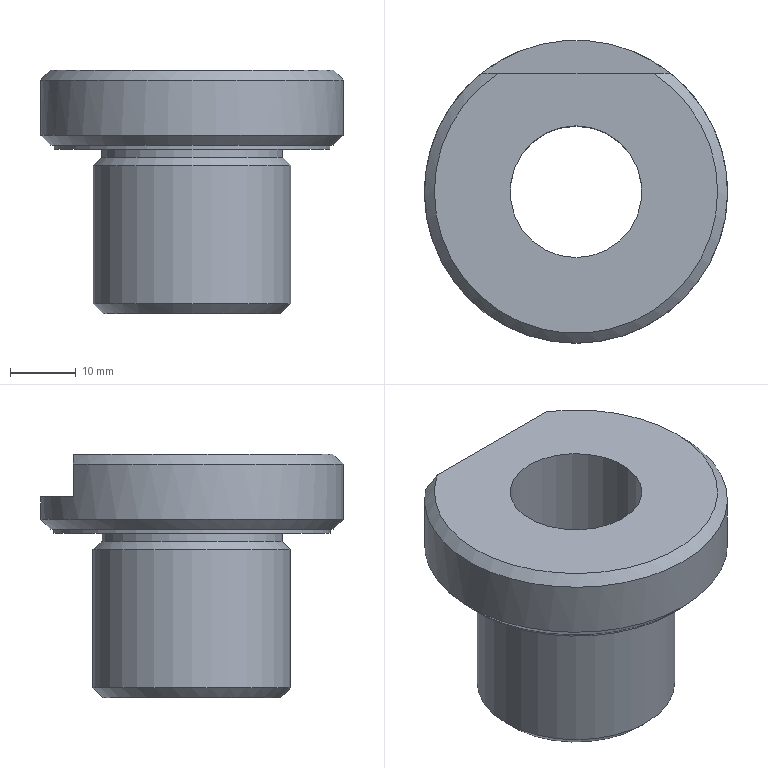Component | NX | DRILL_BUSHING | 1 solid | 15 faces | box 46 x 46 x 37 mm | volume 24582 mm3 | plane 6 | cylinder 5 | cone 4 | commonest cylinder face diameters 46 x1 42 x1 27.5 x1 30 x1 20 x1
STEP:
#1=CARTESIAN_POINT('',(0.,0.,0.));
#2=DIRECTION('',(0.,0.,1.));
#3=DIRECTION('',(1.,0.,0.));
#4=AXIS2_PLACEMENT_3D('',#1,#2,#3);
#5=CARTESIAN_POINT('',(124.,-23.,102.125));
#6=VERTEX_POINT('',#5);
#7=CARTESIAN_POINT('',(124.,0.,102.125));
#8=DIRECTION('',(0.,-0.,-1.));
#9=DIRECTION('',(0.,-1.,0.));
#10=AXIS2_PLACEMENT_3D('',#7,#8,#9);
#11=CIRCLE('',#10,23.);
#12=CARTESIAN_POINT('',(124.,0.,119.5));
#13=DIRECTION('',(0.,-0.,-1.));
#14=DIRECTION('',(0.,-1.,0.));
#15=AXIS2_PLACEMENT_3D('',#12,#13,#14);
#16=CYLINDRICAL_SURFACE('',#15,23.);
#17=CARTESIAN_POINT('',(0.,17.375));
#18=DIRECTION('',(1.,0.));
#19=VECTOR('',#18,1.);
#20=LINE('',#17,#19);
#21=(GEOMETRIC_REPRESENTATION_CONTEXT(2)PARAMETRIC_REPRESENTATION_CONTEXT()REPRESENTATION_CONTEXT('',''));
#22=DEFINITIONAL_REPRESENTATION('',(#20),#21);
#23=PCURVE('',#16,#22);
#24=CARTESIAN_POINT('',(124.,0.,102.125));
#25=DIRECTION('',(0.,0.,1.));
#26=DIRECTION('',(0.,1.,-0.));
#27=AXIS2_PLACEMENT_3D('',#24,#25,#26);
#28=CONICAL_SURFACE('',#27,23.,0.7854);
#29=CARTESIAN_POINT('',(9.425,0.));
#30=DIRECTION('',(-1.,0.));
#31=VECTOR('',#30,1.);
#32=LINE('',#29,#31);
#33=(GEOMETRIC_REPRESENTATION_CONTEXT(2)PARAMETRIC_REPRESENTATION_CONTEXT()REPRESENTATION_CONTEXT('',''));
#34=DEFINITIONAL_REPRESENTATION('',(#32),#33);
#35=PCURVE('',#28,#34);
#36=SURFACE_CURVE('',#11,(#23,#35),.PCURVE_S1.);
#37=EDGE_CURVE('',#6,#6,#36,.T.);
#38=ORIENTED_EDGE('',*,*,#37,.F.);
#39=CARTESIAN_POINT('',(124.,-23.,110.5));
#40=VERTEX_POINT('',#39);
#41=CARTESIAN_POINT('',(124.,-23.,110.5));
#42=CARTESIAN_POINT('',(124.,-23.,102.125));
#43=B_SPLINE_CURVE_WITH_KNOTS('',1,(#41,#42),.UNSPECIFIED.,.F.,.F.,(2,2),(9.,17.375),.PIECEWISE_BEZIER_KNOTS.);
#44=CARTESIAN_POINT('',(0.,0.));
#45=DIRECTION('',(0.,1.));
#46=VECTOR('',#45,1.);
#47=LINE('',#44,#46);
#48=(GEOMETRIC_REPRESENTATION_CONTEXT(2)PARAMETRIC_REPRESENTATION_CONTEXT()REPRESENTATION_CONTEXT('',''));
#49=DEFINITIONAL_REPRESENTATION('',(#47),#48);
#50=PCURVE('',#16,#49);
#51=CARTESIAN_POINT('',(6.283,0.));
#52=DIRECTION('',(0.,1.));
#53=VECTOR('',#52,1.);
#54=LINE('',#51,#53);
#55=(GEOMETRIC_REPRESENTATION_CONTEXT(2)PARAMETRIC_REPRESENTATION_CONTEXT()REPRESENTATION_CONTEXT('',''));
#56=DEFINITIONAL_REPRESENTATION('',(#54),#55);
#57=PCURVE('',#16,#56);
#58=SEAM_CURVE('',#43,(#50,#57),.PCURVE_S1.);
#59=EDGE_CURVE('',#40,#6,#58,.T.);
#60=ORIENTED_EDGE('',*,*,#59,.F.);
#61=CARTESIAN_POINT('',(109.682,18.,110.5));
#62=VERTEX_POINT('',#61);
#63=CARTESIAN_POINT('',(124.,0.,110.5));
#64=DIRECTION('',(0.,-0.,-1.));
#65=DIRECTION('',(0.,-1.,0.));
#66=AXIS2_PLACEMENT_3D('',#63,#64,#65);
#67=CIRCLE('',#66,23.);
#68=CARTESIAN_POINT('',(-6.283,9.));
#69=DIRECTION('',(1.,0.));
#70=VECTOR('',#69,1.);
#71=LINE('',#68,#70);
#72=(GEOMETRIC_REPRESENTATION_CONTEXT(2)PARAMETRIC_REPRESENTATION_CONTEXT()REPRESENTATION_CONTEXT('',''));
#73=DEFINITIONAL_REPRESENTATION('',(#71),#72);
#74=PCURVE('',#16,#73);
#75=CARTESIAN_POINT('',(124.,0.,112.));
#76=DIRECTION('',(0.,-0.,-1.));
#77=DIRECTION('',(0.,-1.,0.));
#78=AXIS2_PLACEMENT_3D('',#75,#76,#77);
#79=CONICAL_SURFACE('',#78,21.5,0.7854);
#80=CARTESIAN_POINT('',(0.,1.5));
#81=DIRECTION('',(1.,0.));
#82=VECTOR('',#81,1.);
#83=LINE('',#80,#82);
#84=(GEOMETRIC_REPRESENTATION_CONTEXT(2)PARAMETRIC_REPRESENTATION_CONTEXT()REPRESENTATION_CONTEXT('',''));
#85=DEFINITIONAL_REPRESENTATION('',(#83),#84);
#86=PCURVE('',#79,#85);
#87=SURFACE_CURVE('',#67,(#74,#86),.PCURVE_S1.);
#88=EDGE_CURVE('',#40,#62,#87,.T.);
#89=ORIENTED_EDGE('',*,*,#88,.T.);
#90=CARTESIAN_POINT('',(109.682,18.,105.5));
#91=VERTEX_POINT('',#90);
#92=CARTESIAN_POINT('',(109.682,18.,119.5));
#93=DIRECTION('',(0.,-0.,-1.));
#94=VECTOR('',#93,1.);
#95=LINE('',#92,#94);
#96=CARTESIAN_POINT('',(2.47,0.));
#97=DIRECTION('',(0.,1.));
#98=VECTOR('',#97,1.);
#99=LINE('',#96,#98);
#100=(GEOMETRIC_REPRESENTATION_CONTEXT(2)PARAMETRIC_REPRESENTATION_CONTEXT()REPRESENTATION_CONTEXT('',''));
#101=DEFINITIONAL_REPRESENTATION('',(#99),#100);
#102=PCURVE('',#16,#101);
#103=CARTESIAN_POINT('',(149.,18.,105.5));
#104=DIRECTION('',(0.,-1.,0.));
#105=DIRECTION('',(0.,0.,1.));
#106=AXIS2_PLACEMENT_3D('',#103,#104,#105);
#107=PLANE('',#106);
#108=CARTESIAN_POINT('',(14.,39.318));
#109=DIRECTION('',(-1.,0.));
#110=VECTOR('',#109,1.);
#111=LINE('',#108,#110);
#112=(GEOMETRIC_REPRESENTATION_CONTEXT(2)PARAMETRIC_REPRESENTATION_CONTEXT()REPRESENTATION_CONTEXT('',''));
#113=DEFINITIONAL_REPRESENTATION('',(#111),#112);
#114=PCURVE('',#107,#113);
#115=SURFACE_CURVE('',#95,(#102,#114),.PCURVE_S1.);
#116=EDGE_CURVE('',#62,#91,#115,.T.);
#117=ORIENTED_EDGE('',*,*,#116,.T.);
#118=CARTESIAN_POINT('',(138.318,18.,105.5));
#119=VERTEX_POINT('',#118);
#120=CARTESIAN_POINT('',(124.,0.,105.5));
#121=DIRECTION('',(0.,-0.,-1.));
#122=DIRECTION('',(0.,-1.,0.));
#123=AXIS2_PLACEMENT_3D('',#120,#121,#122);
#124=CIRCLE('',#123,23.);
#125=CARTESIAN_POINT('',(0.,14.));
#126=DIRECTION('',(1.,0.));
#127=VECTOR('',#126,1.);
#128=LINE('',#125,#127);
#129=(GEOMETRIC_REPRESENTATION_CONTEXT(2)PARAMETRIC_REPRESENTATION_CONTEXT()REPRESENTATION_CONTEXT('',''));
#130=DEFINITIONAL_REPRESENTATION('',(#128),#129);
#131=PCURVE('',#16,#130);
#132=CARTESIAN_POINT('',(149.,39.,105.5));
#133=DIRECTION('',(0.,-0.,-1.));
#134=DIRECTION('',(0.,-1.,0.));
#135=AXIS2_PLACEMENT_3D('',#132,#133,#134);
#136=PLANE('',#135);
#137=CARTESIAN_POINT('',(39.,25.));
#138=DIRECTION('',(1.,0.));
#139=AXIS2_PLACEMENT_2D('',#137,#138);
#140=CIRCLE('',#139,23.);
#141=(GEOMETRIC_REPRESENTATION_CONTEXT(2)PARAMETRIC_REPRESENTATION_CONTEXT()REPRESENTATION_CONTEXT('',''));
#142=DEFINITIONAL_REPRESENTATION('',(#140),#141);
#143=PCURVE('',#136,#142);
#144=SURFACE_CURVE('',#124,(#131,#143),.PCURVE_S1.);
#145=EDGE_CURVE('',#91,#119,#144,.T.);
#146=ORIENTED_EDGE('',*,*,#145,.T.);
#147=CARTESIAN_POINT('',(138.318,18.,110.5));
#148=VERTEX_POINT('',#147);
#149=CARTESIAN_POINT('',(138.318,18.,119.5));
#150=DIRECTION('',(0.,0.,1.));
#151=VECTOR('',#150,1.);
#152=LINE('',#149,#151);
#153=CARTESIAN_POINT('',(3.814,0.));
#154=DIRECTION('',(0.,-1.));
#155=VECTOR('',#154,1.);
#156=LINE('',#153,#155);
#157=(GEOMETRIC_REPRESENTATION_CONTEXT(2)PARAMETRIC_REPRESENTATION_CONTEXT()REPRESENTATION_CONTEXT('',''));
#158=DEFINITIONAL_REPRESENTATION('',(#156),#157);
#159=PCURVE('',#16,#158);
#160=CARTESIAN_POINT('',(14.,10.682));
#161=DIRECTION('',(1.,0.));
#162=VECTOR('',#161,1.);
#163=LINE('',#160,#162);
#164=(GEOMETRIC_REPRESENTATION_CONTEXT(2)PARAMETRIC_REPRESENTATION_CONTEXT()REPRESENTATION_CONTEXT('',''));
#165=DEFINITIONAL_REPRESENTATION('',(#163),#164);
#166=PCURVE('',#107,#165);
#167=SURFACE_CURVE('',#152,(#159,#166),.PCURVE_S1.);
#168=EDGE_CURVE('',#119,#148,#167,.T.);
#169=ORIENTED_EDGE('',*,*,#168,.T.);
#170=CARTESIAN_POINT('',(124.,0.,110.5));
#171=DIRECTION('',(0.,-0.,-1.));
#172=DIRECTION('',(0.,-1.,0.));
#173=AXIS2_PLACEMENT_3D('',#170,#171,#172);
#174=CIRCLE('',#173,23.);
#175=CARTESIAN_POINT('',(0.,9.));
#176=DIRECTION('',(1.,0.));
#177=VECTOR('',#176,1.);
#178=LINE('',#175,#177);
#179=(GEOMETRIC_REPRESENTATION_CONTEXT(2)PARAMETRIC_REPRESENTATION_CONTEXT()REPRESENTATION_CONTEXT('',''));
#180=DEFINITIONAL_REPRESENTATION('',(#178),#179);
#181=PCURVE('',#16,#180);
#182=CARTESIAN_POINT('',(0.,1.5));
#183=DIRECTION('',(1.,-0.));
#184=VECTOR('',#183,1.);
#185=LINE('',#182,#184);
#186=(GEOMETRIC_REPRESENTATION_CONTEXT(2)PARAMETRIC_REPRESENTATION_CONTEXT()REPRESENTATION_CONTEXT('',''));
#187=DEFINITIONAL_REPRESENTATION('',(#185),#186);
#188=PCURVE('',#79,#187);
#189=SURFACE_CURVE('',#174,(#181,#188),.PCURVE_S1.);
#190=EDGE_CURVE('',#148,#40,#189,.T.);
#191=ORIENTED_EDGE('',*,*,#190,.T.);
#192=ORIENTED_EDGE('',*,*,#59,.T.);
#193=EDGE_LOOP('',(#38,#60,#89,#117,#146,#169,#191,#192));
#194=FACE_BOUND('',#193,.T.);
#195=ADVANCED_FACE('',(#194),#16,.T.);
#196=CARTESIAN_POINT('',(124.,-21.5,100.625));
#197=VERTEX_POINT('',#196);
#198=CARTESIAN_POINT('',(124.,-0.,100.625));
#199=DIRECTION('',(0.,-0.,-1.));
#200=DIRECTION('',(0.,-1.,0.));
#201=AXIS2_PLACEMENT_3D('',#198,#199,#200);
#202=CIRCLE('',#201,21.5);
#203=CARTESIAN_POINT('',(9.425,-1.5));
#204=DIRECTION('',(-1.,0.));
#205=VECTOR('',#204,1.);
#206=LINE('',#203,#205);
#207=(GEOMETRIC_REPRESENTATION_CONTEXT(2)PARAMETRIC_REPRESENTATION_CONTEXT()REPRESENTATION_CONTEXT('',''));
#208=DEFINITIONAL_REPRESENTATION('',(#206),#207);
#209=PCURVE('',#28,#208);
#210=CARTESIAN_POINT('',(124.,21.5,100.625));
#211=DIRECTION('',(0.,0.,1.));
#212=DIRECTION('',(0.,1.,-0.));
#213=AXIS2_PLACEMENT_3D('',#210,#211,#212);
#214=PLANE('',#213);
#215=CARTESIAN_POINT('',(-43.,0.));
#216=CARTESIAN_POINT('',(-43.,37.239));
#217=CARTESIAN_POINT('',(-10.75,18.62));
#218=CARTESIAN_POINT('',(21.5,0.));
#219=CARTESIAN_POINT('',(-10.75,-18.62));
#220=CARTESIAN_POINT('',(-43.,-37.239));
#221=CARTESIAN_POINT('',(-43.,0.));
#222=(BOUNDED_CURVE()B_SPLINE_CURVE(2,(#215,#216,#217,#218,#219,#220,#221),.UNSPECIFIED.,.T.,.F.)B_SPLINE_CURVE_WITH_KNOTS((1,2,2,2,2,1),(-2.094,0.,2.094,4.189,6.283,8.378),.UNSPECIFIED.)CURVE()GEOMETRIC_REPRESENTATION_ITEM()RATIONAL_B_SPLINE_CURVE((1.,0.5,1.,0.5,1.,0.5,1.))REPRESENTATION_ITEM(''));
#223=(GEOMETRIC_REPRESENTATION_CONTEXT(2)PARAMETRIC_REPRESENTATION_CONTEXT()REPRESENTATION_CONTEXT('',''));
#224=DEFINITIONAL_REPRESENTATION('',(#222),#223);
#225=PCURVE('',#214,#224);
#226=SURFACE_CURVE('',#202,(#209,#225),.PCURVE_S1.);
#227=EDGE_CURVE('',#197,#197,#226,.T.);
#228=ORIENTED_EDGE('',*,*,#227,.F.);
#229=CARTESIAN_POINT('',(124.,-21.5,100.625));
#230=CARTESIAN_POINT('',(124.,-23.,102.125));
#231=B_SPLINE_CURVE_WITH_KNOTS('',1,(#229,#230),.UNSPECIFIED.,.F.,.F.,(2,2),(-2.121,0.),.PIECEWISE_BEZIER_KNOTS.);
#232=CARTESIAN_POINT('',(9.425,0.));
#233=DIRECTION('',(0.,1.));
#234=VECTOR('',#233,1.);
#235=LINE('',#232,#234);
#236=(GEOMETRIC_REPRESENTATION_CONTEXT(2)PARAMETRIC_REPRESENTATION_CONTEXT()REPRESENTATION_CONTEXT('',''));
#237=DEFINITIONAL_REPRESENTATION('',(#235),#236);
#238=PCURVE('',#28,#237);
#239=CARTESIAN_POINT('',(3.142,0.));
#240=DIRECTION('',(0.,1.));
#241=VECTOR('',#240,1.);
#242=LINE('',#239,#241);
#243=(GEOMETRIC_REPRESENTATION_CONTEXT(2)PARAMETRIC_REPRESENTATION_CONTEXT()REPRESENTATION_CONTEXT('',''));
#244=DEFINITIONAL_REPRESENTATION('',(#242),#243);
#245=PCURVE('',#28,#244);
#246=SEAM_CURVE('',#231,(#238,#245),.PCURVE_S1.);
#247=EDGE_CURVE('',#197,#6,#246,.T.);
#248=ORIENTED_EDGE('',*,*,#247,.T.);
#249=ORIENTED_EDGE('',*,*,#37,.T.);
#250=ORIENTED_EDGE('',*,*,#247,.F.);
#251=EDGE_LOOP('',(#228,#248,#249,#250));
#252=FACE_BOUND('',#251,.T.);
#253=ADVANCED_FACE('',(#252),#28,.T.);
#254=CARTESIAN_POINT('',(124.,-21.,100.625));
#255=VERTEX_POINT('',#254);
#256=CARTESIAN_POINT('',(124.,-0.,100.625));
#257=DIRECTION('',(0.,-0.,-1.));
#258=DIRECTION('',(0.,-1.,0.));
#259=AXIS2_PLACEMENT_3D('',#256,#257,#258);
#260=CIRCLE('',#259,21.);
#261=CARTESIAN_POINT('',(-42.5,0.));
#262=CARTESIAN_POINT('',(-42.5,36.373));
#263=CARTESIAN_POINT('',(-11.,18.187));
#264=CARTESIAN_POINT('',(20.5,0.));
#265=CARTESIAN_POINT('',(-11.,-18.187));
#266=CARTESIAN_POINT('',(-42.5,-36.373));
#267=CARTESIAN_POINT('',(-42.5,0.));
#268=(BOUNDED_CURVE()B_SPLINE_CURVE(2,(#261,#262,#263,#264,#265,#266,#267),.UNSPECIFIED.,.T.,.F.)B_SPLINE_CURVE_WITH_KNOTS((1,2,2,2,2,1),(-2.094,0.,2.094,4.189,6.283,8.378),.UNSPECIFIED.)CURVE()GEOMETRIC_REPRESENTATION_ITEM()RATIONAL_B_SPLINE_CURVE((1.,0.5,1.,0.5,1.,0.5,1.))REPRESENTATION_ITEM(''));
#269=(GEOMETRIC_REPRESENTATION_CONTEXT(2)PARAMETRIC_REPRESENTATION_CONTEXT()REPRESENTATION_CONTEXT('',''));
#270=DEFINITIONAL_REPRESENTATION('',(#268),#269);
#271=PCURVE('',#214,#270);
#272=CARTESIAN_POINT('',(124.,0.,119.5));
#273=DIRECTION('',(0.,-0.,-1.));
#274=DIRECTION('',(0.,-1.,0.));
#275=AXIS2_PLACEMENT_3D('',#272,#273,#274);
#276=CYLINDRICAL_SURFACE('',#275,21.);
#277=CARTESIAN_POINT('',(0.,18.875));
#278=DIRECTION('',(1.,0.));
#279=VECTOR('',#278,1.);
#280=LINE('',#277,#279);
#281=(GEOMETRIC_REPRESENTATION_CONTEXT(2)PARAMETRIC_REPRESENTATION_CONTEXT()REPRESENTATION_CONTEXT('',''));
#282=DEFINITIONAL_REPRESENTATION('',(#280),#281);
#283=PCURVE('',#276,#282);
#284=SURFACE_CURVE('',#260,(#271,#283),.PCURVE_S1.);
#285=EDGE_CURVE('',#255,#255,#284,.T.);
#286=ORIENTED_EDGE('',*,*,#285,.F.);
#287=EDGE_LOOP('',(#286));
#288=FACE_BOUND('',#287,.T.);
#289=ORIENTED_EDGE('',*,*,#227,.T.);
#290=EDGE_LOOP('',(#289));
#291=FACE_BOUND('',#290,.T.);
#292=ADVANCED_FACE('',(#288,#291),#214,.F.);
#293=CARTESIAN_POINT('',(124.,-21.,100.));
#294=VERTEX_POINT('',#293);
#295=CARTESIAN_POINT('',(124.,-0.,100.));
#296=DIRECTION('',(0.,-0.,-1.));
#297=DIRECTION('',(0.,-1.,0.));
#298=AXIS2_PLACEMENT_3D('',#295,#296,#297);
#299=CIRCLE('',#298,21.);
#300=CARTESIAN_POINT('',(0.,19.5));
#301=DIRECTION('',(1.,0.));
#302=VECTOR('',#301,1.);
#303=LINE('',#300,#302);
#304=(GEOMETRIC_REPRESENTATION_CONTEXT(2)PARAMETRIC_REPRESENTATION_CONTEXT()REPRESENTATION_CONTEXT('',''));
#305=DEFINITIONAL_REPRESENTATION('',(#303),#304);
#306=PCURVE('',#276,#305);
#307=CARTESIAN_POINT('',(124.,21.,100.));
#308=DIRECTION('',(0.,0.,1.));
#309=DIRECTION('',(0.,1.,-0.));
#310=AXIS2_PLACEMENT_3D('',#307,#308,#309);
#311=PLANE('',#310);
#312=CARTESIAN_POINT('',(-42.,0.));
#313=CARTESIAN_POINT('',(-42.,36.373));
#314=CARTESIAN_POINT('',(-10.5,18.187));
#315=CARTESIAN_POINT('',(21.,0.));
#316=CARTESIAN_POINT('',(-10.5,-18.187));
#317=CARTESIAN_POINT('',(-42.,-36.373));
#318=CARTESIAN_POINT('',(-42.,0.));
#319=(BOUNDED_CURVE()B_SPLINE_CURVE(2,(#312,#313,#314,#315,#316,#317,#318),.UNSPECIFIED.,.T.,.F.)B_SPLINE_CURVE_WITH_KNOTS((1,2,2,2,2,1),(-2.094,0.,2.094,4.189,6.283,8.378),.UNSPECIFIED.)CURVE()GEOMETRIC_REPRESENTATION_ITEM()RATIONAL_B_SPLINE_CURVE((1.,0.5,1.,0.5,1.,0.5,1.))REPRESENTATION_ITEM(''));
#320=(GEOMETRIC_REPRESENTATION_CONTEXT(2)PARAMETRIC_REPRESENTATION_CONTEXT()REPRESENTATION_CONTEXT('',''));
#321=DEFINITIONAL_REPRESENTATION('',(#319),#320);
#322=PCURVE('',#311,#321);
#323=SURFACE_CURVE('',#299,(#306,#322),.PCURVE_S1.);
#324=EDGE_CURVE('',#294,#294,#323,.T.);
#325=ORIENTED_EDGE('',*,*,#324,.F.);
#326=CARTESIAN_POINT('',(124.,-21.,100.625));
#327=CARTESIAN_POINT('',(124.,-21.,100.));
#328=B_SPLINE_CURVE_WITH_KNOTS('',1,(#326,#327),.UNSPECIFIED.,.F.,.F.,(2,2),(18.875,19.5),.PIECEWISE_BEZIER_KNOTS.);
#329=CARTESIAN_POINT('',(0.,0.));
#330=DIRECTION('',(0.,1.));
#331=VECTOR('',#330,1.);
#332=LINE('',#329,#331);
#333=(GEOMETRIC_REPRESENTATION_CONTEXT(2)PARAMETRIC_REPRESENTATION_CONTEXT()REPRESENTATION_CONTEXT('',''));
#334=DEFINITIONAL_REPRESENTATION('',(#332),#333);
#335=PCURVE('',#276,#334);
#336=CARTESIAN_POINT('',(6.283,0.));
#337=DIRECTION('',(0.,1.));
#338=VECTOR('',#337,1.);
#339=LINE('',#336,#338);
#340=(GEOMETRIC_REPRESENTATION_CONTEXT(2)PARAMETRIC_REPRESENTATION_CONTEXT()REPRESENTATION_CONTEXT('',''));
#341=DEFINITIONAL_REPRESENTATION('',(#339),#340);
#342=PCURVE('',#276,#341);
#343=SEAM_CURVE('',#328,(#335,#342),.PCURVE_S1.);
#344=EDGE_CURVE('',#255,#294,#343,.T.);
#345=ORIENTED_EDGE('',*,*,#344,.F.);
#346=ORIENTED_EDGE('',*,*,#285,.T.);
#347=ORIENTED_EDGE('',*,*,#344,.T.);
#348=EDGE_LOOP('',(#325,#345,#346,#347));
#349=FACE_BOUND('',#348,.T.);
#350=ADVANCED_FACE('',(#349),#276,.T.);
#351=CARTESIAN_POINT('',(124.,-13.75,100.));
#352=VERTEX_POINT('',#351);
#353=CARTESIAN_POINT('',(124.,-0.,100.));
#354=DIRECTION('',(0.,-0.,-1.));
#355=DIRECTION('',(0.,-1.,0.));
#356=AXIS2_PLACEMENT_3D('',#353,#354,#355);
#357=CIRCLE('',#356,13.75);
#358=CARTESIAN_POINT('',(-34.75,0.));
#359=CARTESIAN_POINT('',(-34.75,23.816));
#360=CARTESIAN_POINT('',(-14.125,11.908));
#361=CARTESIAN_POINT('',(6.5,0.));
#362=CARTESIAN_POINT('',(-14.125,-11.908));
#363=CARTESIAN_POINT('',(-34.75,-23.816));
#364=CARTESIAN_POINT('',(-34.75,0.));
#365=(BOUNDED_CURVE()B_SPLINE_CURVE(2,(#358,#359,#360,#361,#362,#363,#364),.UNSPECIFIED.,.T.,.F.)B_SPLINE_CURVE_WITH_KNOTS((1,2,2,2,2,1),(-2.094,0.,2.094,4.189,6.283,8.378),.UNSPECIFIED.)CURVE()GEOMETRIC_REPRESENTATION_ITEM()RATIONAL_B_SPLINE_CURVE((1.,0.5,1.,0.5,1.,0.5,1.))REPRESENTATION_ITEM(''));
#366=(GEOMETRIC_REPRESENTATION_CONTEXT(2)PARAMETRIC_REPRESENTATION_CONTEXT()REPRESENTATION_CONTEXT('',''));
#367=DEFINITIONAL_REPRESENTATION('',(#365),#366);
#368=PCURVE('',#311,#367);
#369=CARTESIAN_POINT('',(124.,0.,119.5));
#370=DIRECTION('',(0.,-0.,-1.));
#371=DIRECTION('',(0.,-1.,0.));
#372=AXIS2_PLACEMENT_3D('',#369,#370,#371);
#373=CYLINDRICAL_SURFACE('',#372,13.75);
#374=CARTESIAN_POINT('',(0.,19.5));
#375=DIRECTION('',(1.,0.));
#376=VECTOR('',#375,1.);
#377=LINE('',#374,#376);
#378=(GEOMETRIC_REPRESENTATION_CONTEXT(2)PARAMETRIC_REPRESENTATION_CONTEXT()REPRESENTATION_CONTEXT('',''));
#379=DEFINITIONAL_REPRESENTATION('',(#377),#378);
#380=PCURVE('',#373,#379);
#381=SURFACE_CURVE('',#357,(#368,#380),.PCURVE_S1.);
#382=EDGE_CURVE('',#352,#352,#381,.T.);
#383=ORIENTED_EDGE('',*,*,#382,.F.);
#384=EDGE_LOOP('',(#383));
#385=FACE_BOUND('',#384,.T.);
#386=ORIENTED_EDGE('',*,*,#324,.T.);
#387=EDGE_LOOP('',(#386));
#388=FACE_BOUND('',#387,.T.);
#389=ADVANCED_FACE('',(#385,#388),#311,.F.);
#390=CARTESIAN_POINT('',(124.,-13.75,98.75));
#391=VERTEX_POINT('',#390);
#392=CARTESIAN_POINT('',(124.,-0.,98.75));
#393=DIRECTION('',(0.,-0.,-1.));
#394=DIRECTION('',(0.,-1.,0.));
#395=AXIS2_PLACEMENT_3D('',#392,#393,#394);
#396=CIRCLE('',#395,13.75);
#397=CARTESIAN_POINT('',(0.,20.75));
#398=DIRECTION('',(1.,0.));
#399=VECTOR('',#398,1.);
#400=LINE('',#397,#399);
#401=(GEOMETRIC_REPRESENTATION_CONTEXT(2)PARAMETRIC_REPRESENTATION_CONTEXT()REPRESENTATION_CONTEXT('',''));
#402=DEFINITIONAL_REPRESENTATION('',(#400),#401);
#403=PCURVE('',#373,#402);
#404=CARTESIAN_POINT('',(124.,-0.,98.75));
#405=DIRECTION('',(0.,-0.,-1.));
#406=DIRECTION('',(0.,-1.,0.));
#407=AXIS2_PLACEMENT_3D('',#404,#405,#406);
#408=CONICAL_SURFACE('',#407,13.75,0.7854);
#409=CARTESIAN_POINT('',(0.,0.));
#410=DIRECTION('',(1.,0.));
#411=VECTOR('',#410,1.);
#412=LINE('',#409,#411);
#413=(GEOMETRIC_REPRESENTATION_CONTEXT(2)PARAMETRIC_REPRESENTATION_CONTEXT()REPRESENTATION_CONTEXT('',''));
#414=DEFINITIONAL_REPRESENTATION('',(#412),#413);
#415=PCURVE('',#408,#414);
#416=SURFACE_CURVE('',#396,(#403,#415),.PCURVE_S1.);
#417=EDGE_CURVE('',#391,#391,#416,.T.);
#418=ORIENTED_EDGE('',*,*,#417,.F.);
#419=CARTESIAN_POINT('',(124.,-13.75,100.));
#420=CARTESIAN_POINT('',(124.,-13.75,98.75));
#421=B_SPLINE_CURVE_WITH_KNOTS('',1,(#419,#420),.UNSPECIFIED.,.F.,.F.,(2,2),(19.5,20.75),.PIECEWISE_BEZIER_KNOTS.);
#422=CARTESIAN_POINT('',(0.,0.));
#423=DIRECTION('',(0.,1.));
#424=VECTOR('',#423,1.);
#425=LINE('',#422,#424);
#426=(GEOMETRIC_REPRESENTATION_CONTEXT(2)PARAMETRIC_REPRESENTATION_CONTEXT()REPRESENTATION_CONTEXT('',''));
#427=DEFINITIONAL_REPRESENTATION('',(#425),#426);
#428=PCURVE('',#373,#427);
#429=CARTESIAN_POINT('',(6.283,0.));
#430=DIRECTION('',(0.,1.));
#431=VECTOR('',#430,1.);
#432=LINE('',#429,#431);
#433=(GEOMETRIC_REPRESENTATION_CONTEXT(2)PARAMETRIC_REPRESENTATION_CONTEXT()REPRESENTATION_CONTEXT('',''));
#434=DEFINITIONAL_REPRESENTATION('',(#432),#433);
#435=PCURVE('',#373,#434);
#436=SEAM_CURVE('',#421,(#428,#435),.PCURVE_S1.);
#437=EDGE_CURVE('',#352,#391,#436,.T.);
#438=ORIENTED_EDGE('',*,*,#437,.F.);
#439=ORIENTED_EDGE('',*,*,#382,.T.);
#440=ORIENTED_EDGE('',*,*,#437,.T.);
#441=EDGE_LOOP('',(#418,#438,#439,#440));
#442=FACE_BOUND('',#441,.T.);
#443=ADVANCED_FACE('',(#442),#373,.T.);
#444=CARTESIAN_POINT('',(124.,-15.,97.5));
#445=VERTEX_POINT('',#444);
#446=CARTESIAN_POINT('',(124.,-0.,97.5));
#447=DIRECTION('',(0.,-0.,-1.));
#448=DIRECTION('',(0.,-1.,0.));
#449=AXIS2_PLACEMENT_3D('',#446,#447,#448);
#450=CIRCLE('',#449,15.);
#451=CARTESIAN_POINT('',(0.,1.25));
#452=DIRECTION('',(1.,0.));
#453=VECTOR('',#452,1.);
#454=LINE('',#451,#453);
#455=(GEOMETRIC_REPRESENTATION_CONTEXT(2)PARAMETRIC_REPRESENTATION_CONTEXT()REPRESENTATION_CONTEXT('',''));
#456=DEFINITIONAL_REPRESENTATION('',(#454),#455);
#457=PCURVE('',#408,#456);
#458=CARTESIAN_POINT('',(124.,0.,119.5));
#459=DIRECTION('',(0.,-0.,-1.));
#460=DIRECTION('',(0.,-1.,0.));
#461=AXIS2_PLACEMENT_3D('',#458,#459,#460);
#462=CYLINDRICAL_SURFACE('',#461,15.);
#463=CARTESIAN_POINT('',(0.,22.));
#464=DIRECTION('',(1.,0.));
#465=VECTOR('',#464,1.);
#466=LINE('',#463,#465);
#467=(GEOMETRIC_REPRESENTATION_CONTEXT(2)PARAMETRIC_REPRESENTATION_CONTEXT()REPRESENTATION_CONTEXT('',''));
#468=DEFINITIONAL_REPRESENTATION('',(#466),#467);
#469=PCURVE('',#462,#468);
#470=SURFACE_CURVE('',#450,(#457,#469),.PCURVE_S1.);
#471=EDGE_CURVE('',#445,#445,#470,.T.);
#472=ORIENTED_EDGE('',*,*,#471,.F.);
#473=CARTESIAN_POINT('',(124.,-13.75,98.75));
#474=CARTESIAN_POINT('',(124.,-15.,97.5));
#475=B_SPLINE_CURVE_WITH_KNOTS('',1,(#473,#474),.UNSPECIFIED.,.F.,.F.,(2,2),(0.,1.768),.PIECEWISE_BEZIER_KNOTS.);
#476=CARTESIAN_POINT('',(0.,0.));
#477=DIRECTION('',(0.,1.));
#478=VECTOR('',#477,1.);
#479=LINE('',#476,#478);
#480=(GEOMETRIC_REPRESENTATION_CONTEXT(2)PARAMETRIC_REPRESENTATION_CONTEXT()REPRESENTATION_CONTEXT('',''));
#481=DEFINITIONAL_REPRESENTATION('',(#479),#480);
#482=PCURVE('',#408,#481);
#483=CARTESIAN_POINT('',(6.283,0.));
#484=DIRECTION('',(0.,1.));
#485=VECTOR('',#484,1.);
#486=LINE('',#483,#485);
#487=(GEOMETRIC_REPRESENTATION_CONTEXT(2)PARAMETRIC_REPRESENTATION_CONTEXT()REPRESENTATION_CONTEXT('',''));
#488=DEFINITIONAL_REPRESENTATION('',(#486),#487);
#489=PCURVE('',#408,#488);
#490=SEAM_CURVE('',#475,(#482,#489),.PCURVE_S1.);
#491=EDGE_CURVE('',#391,#445,#490,.T.);
#492=ORIENTED_EDGE('',*,*,#491,.F.);
#493=ORIENTED_EDGE('',*,*,#417,.T.);
#494=ORIENTED_EDGE('',*,*,#491,.T.);
#495=EDGE_LOOP('',(#472,#492,#493,#494));
#496=FACE_BOUND('',#495,.T.);
#497=ADVANCED_FACE('',(#496),#408,.T.);
#498=CARTESIAN_POINT('',(124.,-15.,76.5));
#499=VERTEX_POINT('',#498);
#500=CARTESIAN_POINT('',(124.,-0.,76.5));
#501=DIRECTION('',(0.,-0.,-1.));
#502=DIRECTION('',(0.,-1.,0.));
#503=AXIS2_PLACEMENT_3D('',#500,#501,#502);
#504=CIRCLE('',#503,15.);
#505=CARTESIAN_POINT('',(0.,43.));
#506=DIRECTION('',(1.,0.));
#507=VECTOR('',#506,1.);
#508=LINE('',#505,#507);
#509=(GEOMETRIC_REPRESENTATION_CONTEXT(2)PARAMETRIC_REPRESENTATION_CONTEXT()REPRESENTATION_CONTEXT('',''));
#510=DEFINITIONAL_REPRESENTATION('',(#508),#509);
#511=PCURVE('',#462,#510);
#512=CARTESIAN_POINT('',(124.,-0.,76.5));
#513=DIRECTION('',(0.,0.,1.));
#514=DIRECTION('',(0.,1.,-0.));
#515=AXIS2_PLACEMENT_3D('',#512,#513,#514);
#516=CONICAL_SURFACE('',#515,15.,0.7854);
#517=CARTESIAN_POINT('',(9.425,0.));
#518=DIRECTION('',(-1.,0.));
#519=VECTOR('',#518,1.);
#520=LINE('',#517,#519);
#521=(GEOMETRIC_REPRESENTATION_CONTEXT(2)PARAMETRIC_REPRESENTATION_CONTEXT()REPRESENTATION_CONTEXT('',''));
#522=DEFINITIONAL_REPRESENTATION('',(#520),#521);
#523=PCURVE('',#516,#522);
#524=SURFACE_CURVE('',#504,(#511,#523),.PCURVE_S1.);
#525=EDGE_CURVE('',#499,#499,#524,.T.);
#526=ORIENTED_EDGE('',*,*,#525,.F.);
#527=CARTESIAN_POINT('',(124.,-15.,97.5));
#528=CARTESIAN_POINT('',(124.,-15.,76.5));
#529=B_SPLINE_CURVE_WITH_KNOTS('',1,(#527,#528),.UNSPECIFIED.,.F.,.F.,(2,2),(22.,43.),.PIECEWISE_BEZIER_KNOTS.);
#530=CARTESIAN_POINT('',(0.,0.));
#531=DIRECTION('',(0.,1.));
#532=VECTOR('',#531,1.);
#533=LINE('',#530,#532);
#534=(GEOMETRIC_REPRESENTATION_CONTEXT(2)PARAMETRIC_REPRESENTATION_CONTEXT()REPRESENTATION_CONTEXT('',''));
#535=DEFINITIONAL_REPRESENTATION('',(#533),#534);
#536=PCURVE('',#462,#535);
#537=CARTESIAN_POINT('',(6.283,0.));
#538=DIRECTION('',(0.,1.));
#539=VECTOR('',#538,1.);
#540=LINE('',#537,#539);
#541=(GEOMETRIC_REPRESENTATION_CONTEXT(2)PARAMETRIC_REPRESENTATION_CONTEXT()REPRESENTATION_CONTEXT('',''));
#542=DEFINITIONAL_REPRESENTATION('',(#540),#541);
#543=PCURVE('',#462,#542);
#544=SEAM_CURVE('',#529,(#536,#543),.PCURVE_S1.);
#545=EDGE_CURVE('',#445,#499,#544,.T.);
#546=ORIENTED_EDGE('',*,*,#545,.F.);
#547=ORIENTED_EDGE('',*,*,#471,.T.);
#548=ORIENTED_EDGE('',*,*,#545,.T.);
#549=EDGE_LOOP('',(#526,#546,#547,#548));
#550=FACE_BOUND('',#549,.T.);
#551=ADVANCED_FACE('',(#550),#462,.T.);
#552=CARTESIAN_POINT('',(124.,-13.5,75.));
#553=VERTEX_POINT('',#552);
#554=CARTESIAN_POINT('',(124.,-0.,75.));
#555=DIRECTION('',(0.,-0.,-1.));
#556=DIRECTION('',(0.,-1.,0.));
#557=AXIS2_PLACEMENT_3D('',#554,#555,#556);
#558=CIRCLE('',#557,13.5);
#559=CARTESIAN_POINT('',(9.425,-1.5));
#560=DIRECTION('',(-1.,0.));
#561=VECTOR('',#560,1.);
#562=LINE('',#559,#561);
#563=(GEOMETRIC_REPRESENTATION_CONTEXT(2)PARAMETRIC_REPRESENTATION_CONTEXT()REPRESENTATION_CONTEXT('',''));
#564=DEFINITIONAL_REPRESENTATION('',(#562),#563);
#565=PCURVE('',#516,#564);
#566=CARTESIAN_POINT('',(124.,13.5,75.));
#567=DIRECTION('',(0.,0.,1.));
#568=DIRECTION('',(0.,1.,-0.));
#569=AXIS2_PLACEMENT_3D('',#566,#567,#568);
#570=PLANE('',#569);
#571=CARTESIAN_POINT('',(-27.,0.));
#572=CARTESIAN_POINT('',(-27.,23.383));
#573=CARTESIAN_POINT('',(-6.75,11.691));
#574=CARTESIAN_POINT('',(13.5,0.));
#575=CARTESIAN_POINT('',(-6.75,-11.691));
#576=CARTESIAN_POINT('',(-27.,-23.383));
#577=CARTESIAN_POINT('',(-27.,0.));
#578=(BOUNDED_CURVE()B_SPLINE_CURVE(2,(#571,#572,#573,#574,#575,#576,#577),.UNSPECIFIED.,.T.,.F.)B_SPLINE_CURVE_WITH_KNOTS((1,2,2,2,2,1),(-2.094,0.,2.094,4.189,6.283,8.378),.UNSPECIFIED.)CURVE()GEOMETRIC_REPRESENTATION_ITEM()RATIONAL_B_SPLINE_CURVE((1.,0.5,1.,0.5,1.,0.5,1.))REPRESENTATION_ITEM(''));
#579=(GEOMETRIC_REPRESENTATION_CONTEXT(2)PARAMETRIC_REPRESENTATION_CONTEXT()REPRESENTATION_CONTEXT('',''));
#580=DEFINITIONAL_REPRESENTATION('',(#578),#579);
#581=PCURVE('',#570,#580);
#582=SURFACE_CURVE('',#558,(#565,#581),.PCURVE_S1.);
#583=EDGE_CURVE('',#553,#553,#582,.T.);
#584=ORIENTED_EDGE('',*,*,#583,.F.);
#585=CARTESIAN_POINT('',(124.,-13.5,75.));
#586=CARTESIAN_POINT('',(124.,-15.,76.5));
#587=B_SPLINE_CURVE_WITH_KNOTS('',1,(#585,#586),.UNSPECIFIED.,.F.,.F.,(2,2),(-2.121,0.),.PIECEWISE_BEZIER_KNOTS.);
#588=CARTESIAN_POINT('',(9.425,0.));
#589=DIRECTION('',(0.,1.));
#590=VECTOR('',#589,1.);
#591=LINE('',#588,#590);
#592=(GEOMETRIC_REPRESENTATION_CONTEXT(2)PARAMETRIC_REPRESENTATION_CONTEXT()REPRESENTATION_CONTEXT('',''));
#593=DEFINITIONAL_REPRESENTATION('',(#591),#592);
#594=PCURVE('',#516,#593);
#595=CARTESIAN_POINT('',(3.142,0.));
#596=DIRECTION('',(0.,1.));
#597=VECTOR('',#596,1.);
#598=LINE('',#595,#597);
#599=(GEOMETRIC_REPRESENTATION_CONTEXT(2)PARAMETRIC_REPRESENTATION_CONTEXT()REPRESENTATION_CONTEXT('',''));
#600=DEFINITIONAL_REPRESENTATION('',(#598),#599);
#601=PCURVE('',#516,#600);
#602=SEAM_CURVE('',#587,(#594,#601),.PCURVE_S1.);
#603=EDGE_CURVE('',#553,#499,#602,.T.);
#604=ORIENTED_EDGE('',*,*,#603,.T.);
#605=ORIENTED_EDGE('',*,*,#525,.T.);
#606=ORIENTED_EDGE('',*,*,#603,.F.);
#607=EDGE_LOOP('',(#584,#604,#605,#606));
#608=FACE_BOUND('',#607,.T.);
#609=ADVANCED_FACE('',(#608),#516,.T.);
#610=CARTESIAN_POINT('',(124.,10.,75.));
#611=VERTEX_POINT('',#610);
#612=CARTESIAN_POINT('',(124.,-0.,75.));
#613=DIRECTION('',(0.,0.,1.));
#614=DIRECTION('',(0.,1.,-0.));
#615=AXIS2_PLACEMENT_3D('',#612,#613,#614);
#616=CIRCLE('',#615,10.);
#617=CARTESIAN_POINT('',(-13.5,0.));
#618=DIRECTION('',(1.,0.));
#619=AXIS2_PLACEMENT_2D('',#617,#618);
#620=CIRCLE('',#619,10.);
#621=(GEOMETRIC_REPRESENTATION_CONTEXT(2)PARAMETRIC_REPRESENTATION_CONTEXT()REPRESENTATION_CONTEXT('',''));
#622=DEFINITIONAL_REPRESENTATION('',(#620),#621);
#623=PCURVE('',#570,#622);
#624=CARTESIAN_POINT('',(124.,-0.,75.));
#625=DIRECTION('',(0.,0.,1.));
#626=DIRECTION('',(0.,1.,-0.));
#627=AXIS2_PLACEMENT_3D('',#624,#625,#626);
#628=CYLINDRICAL_SURFACE('',#627,10.);
#629=CARTESIAN_POINT('',(0.,0.));
#630=DIRECTION('',(1.,0.));
#631=VECTOR('',#630,1.);
#632=LINE('',#629,#631);
#633=(GEOMETRIC_REPRESENTATION_CONTEXT(2)PARAMETRIC_REPRESENTATION_CONTEXT()REPRESENTATION_CONTEXT('',''));
#634=DEFINITIONAL_REPRESENTATION('',(#632),#633);
#635=PCURVE('',#628,#634);
#636=SURFACE_CURVE('',#616,(#623,#635),.PCURVE_S1.);
#637=EDGE_CURVE('',#611,#611,#636,.T.);
#638=ORIENTED_EDGE('',*,*,#637,.T.);
#639=EDGE_LOOP('',(#638));
#640=FACE_BOUND('',#639,.T.);
#641=ORIENTED_EDGE('',*,*,#583,.T.);
#642=EDGE_LOOP('',(#641));
#643=FACE_BOUND('',#642,.T.);
#644=ADVANCED_FACE('',(#640,#643),#570,.F.);
#645=CARTESIAN_POINT('',(124.,-10.,112.));
#646=VERTEX_POINT('',#645);
#647=CARTESIAN_POINT('',(124.,10.,112.));
#648=VERTEX_POINT('',#647);
#649=CARTESIAN_POINT('',(124.,0.,112.));
#650=DIRECTION('',(0.,-0.,-1.));
#651=DIRECTION('',(0.,-1.,0.));
#652=AXIS2_PLACEMENT_3D('',#649,#650,#651);
#653=CIRCLE('',#652,10.);
#654=CARTESIAN_POINT('',(124.,0.,112.));
#655=DIRECTION('',(0.,-0.,-1.));
#656=DIRECTION('',(0.,-1.,0.));
#657=AXIS2_PLACEMENT_3D('',#654,#655,#656);
#658=PLANE('',#657);
#659=CARTESIAN_POINT('',(0.,0.));
#660=DIRECTION('',(1.,0.));
#661=AXIS2_PLACEMENT_2D('',#659,#660);
#662=CIRCLE('',#661,10.);
#663=(GEOMETRIC_REPRESENTATION_CONTEXT(2)PARAMETRIC_REPRESENTATION_CONTEXT()REPRESENTATION_CONTEXT('',''));
#664=DEFINITIONAL_REPRESENTATION('',(#662),#663);
#665=PCURVE('',#658,#664);
#666=CARTESIAN_POINT('',(3.142,37.));
#667=DIRECTION('',(-1.,0.));
#668=VECTOR('',#667,1.);
#669=LINE('',#666,#668);
#670=(GEOMETRIC_REPRESENTATION_CONTEXT(2)PARAMETRIC_REPRESENTATION_CONTEXT()REPRESENTATION_CONTEXT('',''));
#671=DEFINITIONAL_REPRESENTATION('',(#669),#670);
#672=PCURVE('',#628,#671);
#673=SURFACE_CURVE('',#653,(#665,#672),.PCURVE_S1.);
#674=EDGE_CURVE('',#646,#648,#673,.T.);
#675=ORIENTED_EDGE('',*,*,#674,.T.);
#676=CARTESIAN_POINT('',(124.,0.,112.));
#677=DIRECTION('',(0.,-0.,-1.));
#678=DIRECTION('',(0.,-1.,0.));
#679=AXIS2_PLACEMENT_3D('',#676,#677,#678);
#680=CIRCLE('',#679,10.);
#681=CARTESIAN_POINT('',(0.,0.));
#682=DIRECTION('',(1.,0.));
#683=AXIS2_PLACEMENT_2D('',#681,#682);
#684=CIRCLE('',#683,10.);
#685=(GEOMETRIC_REPRESENTATION_CONTEXT(2)PARAMETRIC_REPRESENTATION_CONTEXT()REPRESENTATION_CONTEXT('',''));
#686=DEFINITIONAL_REPRESENTATION('',(#684),#685);
#687=PCURVE('',#658,#686);
#688=CARTESIAN_POINT('',(9.425,37.));
#689=DIRECTION('',(-1.,0.));
#690=VECTOR('',#689,1.);
#691=LINE('',#688,#690);
#692=(GEOMETRIC_REPRESENTATION_CONTEXT(2)PARAMETRIC_REPRESENTATION_CONTEXT()REPRESENTATION_CONTEXT('',''));
#693=DEFINITIONAL_REPRESENTATION('',(#691),#692);
#694=PCURVE('',#628,#693);
#695=SURFACE_CURVE('',#680,(#687,#694),.PCURVE_S1.);
#696=EDGE_CURVE('',#648,#646,#695,.T.);
#697=ORIENTED_EDGE('',*,*,#696,.T.);
#698=EDGE_LOOP('',(#675,#697));
#699=FACE_BOUND('',#698,.T.);
#700=CARTESIAN_POINT('',(135.758,18.,112.));
#701=VERTEX_POINT('',#700);
#702=CARTESIAN_POINT('',(112.242,18.,112.));
#703=VERTEX_POINT('',#702);
#704=CARTESIAN_POINT('',(124.,0.,112.));
#705=DIRECTION('',(0.,-0.,-1.));
#706=DIRECTION('',(0.,-1.,0.));
#707=AXIS2_PLACEMENT_3D('',#704,#705,#706);
#708=CIRCLE('',#707,21.5);
#709=CARTESIAN_POINT('',(0.,0.));
#710=DIRECTION('',(1.,0.));
#711=AXIS2_PLACEMENT_2D('',#709,#710);
#712=CIRCLE('',#711,21.5);
#713=(GEOMETRIC_REPRESENTATION_CONTEXT(2)PARAMETRIC_REPRESENTATION_CONTEXT()REPRESENTATION_CONTEXT('',''));
#714=DEFINITIONAL_REPRESENTATION('',(#712),#713);
#715=PCURVE('',#658,#714);
#716=CARTESIAN_POINT('',(-0.,-0.));
#717=DIRECTION('',(1.,0.));
#718=VECTOR('',#717,1.);
#719=LINE('',#716,#718);
#720=(GEOMETRIC_REPRESENTATION_CONTEXT(2)PARAMETRIC_REPRESENTATION_CONTEXT()REPRESENTATION_CONTEXT('',''));
#721=DEFINITIONAL_REPRESENTATION('',(#719),#720);
#722=PCURVE('',#79,#721);
#723=SURFACE_CURVE('',#708,(#715,#722),.PCURVE_S1.);
#724=EDGE_CURVE('',#701,#703,#723,.T.);
#725=ORIENTED_EDGE('',*,*,#724,.F.);
#726=CARTESIAN_POINT('',(124.,18.,112.));
#727=DIRECTION('',(-1.,0.,0.));
#728=VECTOR('',#727,1.);
#729=LINE('',#726,#728);
#730=CARTESIAN_POINT('',(-18.,0.));
#731=DIRECTION('',(0.,1.));
#732=VECTOR('',#731,1.);
#733=LINE('',#730,#732);
#734=(GEOMETRIC_REPRESENTATION_CONTEXT(2)PARAMETRIC_REPRESENTATION_CONTEXT()REPRESENTATION_CONTEXT('',''));
#735=DEFINITIONAL_REPRESENTATION('',(#733),#734);
#736=PCURVE('',#658,#735);
#737=CARTESIAN_POINT('',(6.5,25.));
#738=DIRECTION('',(0.,1.));
#739=VECTOR('',#738,1.);
#740=LINE('',#737,#739);
#741=(GEOMETRIC_REPRESENTATION_CONTEXT(2)PARAMETRIC_REPRESENTATION_CONTEXT()REPRESENTATION_CONTEXT('',''));
#742=DEFINITIONAL_REPRESENTATION('',(#740),#741);
#743=PCURVE('',#107,#742);
#744=SURFACE_CURVE('',#729,(#736,#743),.PCURVE_S1.);
#745=EDGE_CURVE('',#701,#703,#744,.T.);
#746=ORIENTED_EDGE('',*,*,#745,.T.);
#747=EDGE_LOOP('',(#725,#746));
#748=FACE_BOUND('',#747,.T.);
#749=ADVANCED_FACE('',(#699,#748),#658,.F.);
#750=ORIENTED_EDGE('',*,*,#190,.F.);
#751=CARTESIAN_POINT('',(138.318,18.,110.5));
#752=CARTESIAN_POINT('',(137.478,18.,111.023));
#753=CARTESIAN_POINT('',(136.624,18.,111.526));
#754=CARTESIAN_POINT('',(135.758,18.,112.));
#755=B_SPLINE_CURVE_WITH_KNOTS('',3,(#751,#752,#753,#754),.UNSPECIFIED.,.F.,.F.,(4,4),(0.,1.),.PIECEWISE_BEZIER_KNOTS.);
#756=CARTESIAN_POINT('',(3.814,1.5));
#757=CARTESIAN_POINT('',(3.72,0.));
#758=B_SPLINE_CURVE_WITH_KNOTS('',1,(#756,#757),.UNSPECIFIED.,.F.,.F.,(2,2),(0.,1.),.PIECEWISE_BEZIER_KNOTS.);
#759=(GEOMETRIC_REPRESENTATION_CONTEXT(2)PARAMETRIC_REPRESENTATION_CONTEXT()REPRESENTATION_CONTEXT('',''));
#760=DEFINITIONAL_REPRESENTATION('',(#758),#759);
#761=PCURVE('',#79,#760);
#762=CARTESIAN_POINT('',(5.,10.682));
#763=CARTESIAN_POINT('',(5.523,11.522));
#764=CARTESIAN_POINT('',(6.026,12.376));
#765=CARTESIAN_POINT('',(6.5,13.242));
#766=B_SPLINE_CURVE_WITH_KNOTS('',3,(#762,#763,#764,#765),.UNSPECIFIED.,.F.,.F.,(4,4),(0.,1.),.PIECEWISE_BEZIER_KNOTS.);
#767=(GEOMETRIC_REPRESENTATION_CONTEXT(2)PARAMETRIC_REPRESENTATION_CONTEXT()REPRESENTATION_CONTEXT('',''));
#768=DEFINITIONAL_REPRESENTATION('',(#766),#767);
#769=PCURVE('',#107,#768);
#770=SURFACE_CURVE('',#755,(#761,#769),.PCURVE_S1.);
#771=EDGE_CURVE('',#148,#701,#770,.T.);
#772=ORIENTED_EDGE('',*,*,#771,.T.);
#773=ORIENTED_EDGE('',*,*,#724,.T.);
#774=CARTESIAN_POINT('',(112.242,18.,112.));
#775=CARTESIAN_POINT('',(111.374,18.,111.525));
#776=CARTESIAN_POINT('',(110.522,18.,111.023));
#777=CARTESIAN_POINT('',(109.682,18.,110.5));
#778=B_SPLINE_CURVE_WITH_KNOTS('',3,(#774,#775,#776,#777),.UNSPECIFIED.,.F.,.F.,(4,4),(0.,1.),.PIECEWISE_BEZIER_KNOTS.);
#779=CARTESIAN_POINT('',(8.846,0.));
#780=CARTESIAN_POINT('',(8.753,1.5));
#781=B_SPLINE_CURVE_WITH_KNOTS('',1,(#779,#780),.UNSPECIFIED.,.F.,.F.,(2,2),(0.,1.),.PIECEWISE_BEZIER_KNOTS.);
#782=(GEOMETRIC_REPRESENTATION_CONTEXT(2)PARAMETRIC_REPRESENTATION_CONTEXT()REPRESENTATION_CONTEXT('',''));
#783=DEFINITIONAL_REPRESENTATION('',(#781),#782);
#784=PCURVE('',#79,#783);
#785=CARTESIAN_POINT('',(6.5,36.758));
#786=CARTESIAN_POINT('',(6.025,37.626));
#787=CARTESIAN_POINT('',(5.523,38.478));
#788=CARTESIAN_POINT('',(5.,39.318));
#789=B_SPLINE_CURVE_WITH_KNOTS('',3,(#785,#786,#787,#788),.UNSPECIFIED.,.F.,.F.,(4,4),(0.,1.),.PIECEWISE_BEZIER_KNOTS.);
#790=(GEOMETRIC_REPRESENTATION_CONTEXT(2)PARAMETRIC_REPRESENTATION_CONTEXT()REPRESENTATION_CONTEXT('',''));
#791=DEFINITIONAL_REPRESENTATION('',(#789),#790);
#792=PCURVE('',#107,#791);
#793=SURFACE_CURVE('',#778,(#784,#792),.PCURVE_S1.);
#794=EDGE_CURVE('',#703,#62,#793,.T.);
#795=ORIENTED_EDGE('',*,*,#794,.T.);
#796=ORIENTED_EDGE('',*,*,#88,.F.);
#797=EDGE_LOOP('',(#750,#772,#773,#795,#796));
#798=FACE_BOUND('',#797,.T.);
#799=ADVANCED_FACE('',(#798),#79,.T.);
#800=ORIENTED_EDGE('',*,*,#637,.T.);
#801=CARTESIAN_POINT('',(124.,10.,75.));
#802=CARTESIAN_POINT('',(124.,10.,112.));
#803=B_SPLINE_CURVE_WITH_KNOTS('',1,(#801,#802),.UNSPECIFIED.,.F.,.F.,(2,2),(0.,37.),.PIECEWISE_BEZIER_KNOTS.);
#804=CARTESIAN_POINT('',(6.283,0.));
#805=DIRECTION('',(0.,1.));
#806=VECTOR('',#805,1.);
#807=LINE('',#804,#806);
#808=(GEOMETRIC_REPRESENTATION_CONTEXT(2)PARAMETRIC_REPRESENTATION_CONTEXT()REPRESENTATION_CONTEXT('',''));
#809=DEFINITIONAL_REPRESENTATION('',(#807),#808);
#810=PCURVE('',#628,#809);
#811=CARTESIAN_POINT('',(0.,0.));
#812=DIRECTION('',(0.,1.));
#813=VECTOR('',#812,1.);
#814=LINE('',#811,#813);
#815=(GEOMETRIC_REPRESENTATION_CONTEXT(2)PARAMETRIC_REPRESENTATION_CONTEXT()REPRESENTATION_CONTEXT('',''));
#816=DEFINITIONAL_REPRESENTATION('',(#814),#815);
#817=PCURVE('',#628,#816);
#818=SEAM_CURVE('',#803,(#810,#817),.PCURVE_S1.);
#819=EDGE_CURVE('',#611,#648,#818,.T.);
#820=ORIENTED_EDGE('',*,*,#819,.T.);
#821=ORIENTED_EDGE('',*,*,#696,.T.);
#822=ORIENTED_EDGE('',*,*,#674,.T.);
#823=ORIENTED_EDGE('',*,*,#819,.F.);
#824=EDGE_LOOP('',(#800,#820,#821,#822,#823));
#825=FACE_BOUND('',#824,.F.);
#826=ADVANCED_FACE('',(#825),#628,.F.);
#827=CARTESIAN_POINT('',(149.,18.,105.5));
#828=DIRECTION('',(1.,0.,0.));
#829=VECTOR('',#828,1.);
#830=LINE('',#827,#829);
#831=CARTESIAN_POINT('',(21.,0.));
#832=DIRECTION('',(0.,-1.));
#833=VECTOR('',#832,1.);
#834=LINE('',#831,#833);
#835=(GEOMETRIC_REPRESENTATION_CONTEXT(2)PARAMETRIC_REPRESENTATION_CONTEXT()REPRESENTATION_CONTEXT('',''));
#836=DEFINITIONAL_REPRESENTATION('',(#834),#835);
#837=PCURVE('',#136,#836);
#838=CARTESIAN_POINT('',(0.,0.));
#839=DIRECTION('',(0.,-1.));
#840=VECTOR('',#839,1.);
#841=LINE('',#838,#840);
#842=(GEOMETRIC_REPRESENTATION_CONTEXT(2)PARAMETRIC_REPRESENTATION_CONTEXT()REPRESENTATION_CONTEXT('',''));
#843=DEFINITIONAL_REPRESENTATION('',(#841),#842);
#844=PCURVE('',#107,#843);
#845=SURFACE_CURVE('',#830,(#837,#844),.PCURVE_S1.);
#846=EDGE_CURVE('',#91,#119,#845,.T.);
#847=ORIENTED_EDGE('',*,*,#846,.T.);
#848=ORIENTED_EDGE('',*,*,#145,.F.);
#849=EDGE_LOOP('',(#847,#848));
#850=FACE_BOUND('',#849,.T.);
#851=ADVANCED_FACE('',(#850),#136,.F.);
#852=ORIENTED_EDGE('',*,*,#846,.F.);
#853=ORIENTED_EDGE('',*,*,#116,.F.);
#854=ORIENTED_EDGE('',*,*,#794,.F.);
#855=ORIENTED_EDGE('',*,*,#745,.F.);
#856=ORIENTED_EDGE('',*,*,#771,.F.);
#857=ORIENTED_EDGE('',*,*,#168,.F.);
#858=EDGE_LOOP('',(#852,#853,#854,#855,#856,#857));
#859=FACE_BOUND('',#858,.T.);
#860=ADVANCED_FACE('',(#859),#107,.F.);
#861=CLOSED_SHELL('',(#195,#253,#292,#350,#389,#443,#497,#551,#609,#644,#749,#799,#826,#851,#860));
#862=MANIFOLD_SOLID_BREP('',#861);
#863=(LENGTH_UNIT()NAMED_UNIT(*)SI_UNIT(.MILLI.,.METRE.));
#864=UNCERTAINTY_MEASURE_WITH_UNIT(LENGTH_MEASURE(0.01),#863,'','');
#865=(NAMED_UNIT(*)PLANE_ANGLE_UNIT()SI_UNIT($,.RADIAN.));
#866=(NAMED_UNIT(*)SI_UNIT($,.STERADIAN.)SOLID_ANGLE_UNIT());
#867=(GEOMETRIC_REPRESENTATION_CONTEXT(3)GLOBAL_UNCERTAINTY_ASSIGNED_CONTEXT((#864))GLOBAL_UNIT_ASSIGNED_CONTEXT((#863,#865,#866))REPRESENTATION_CONTEXT('',''));
#868=ADVANCED_BREP_SHAPE_REPRESENTATION('',(#4,#862),#867);